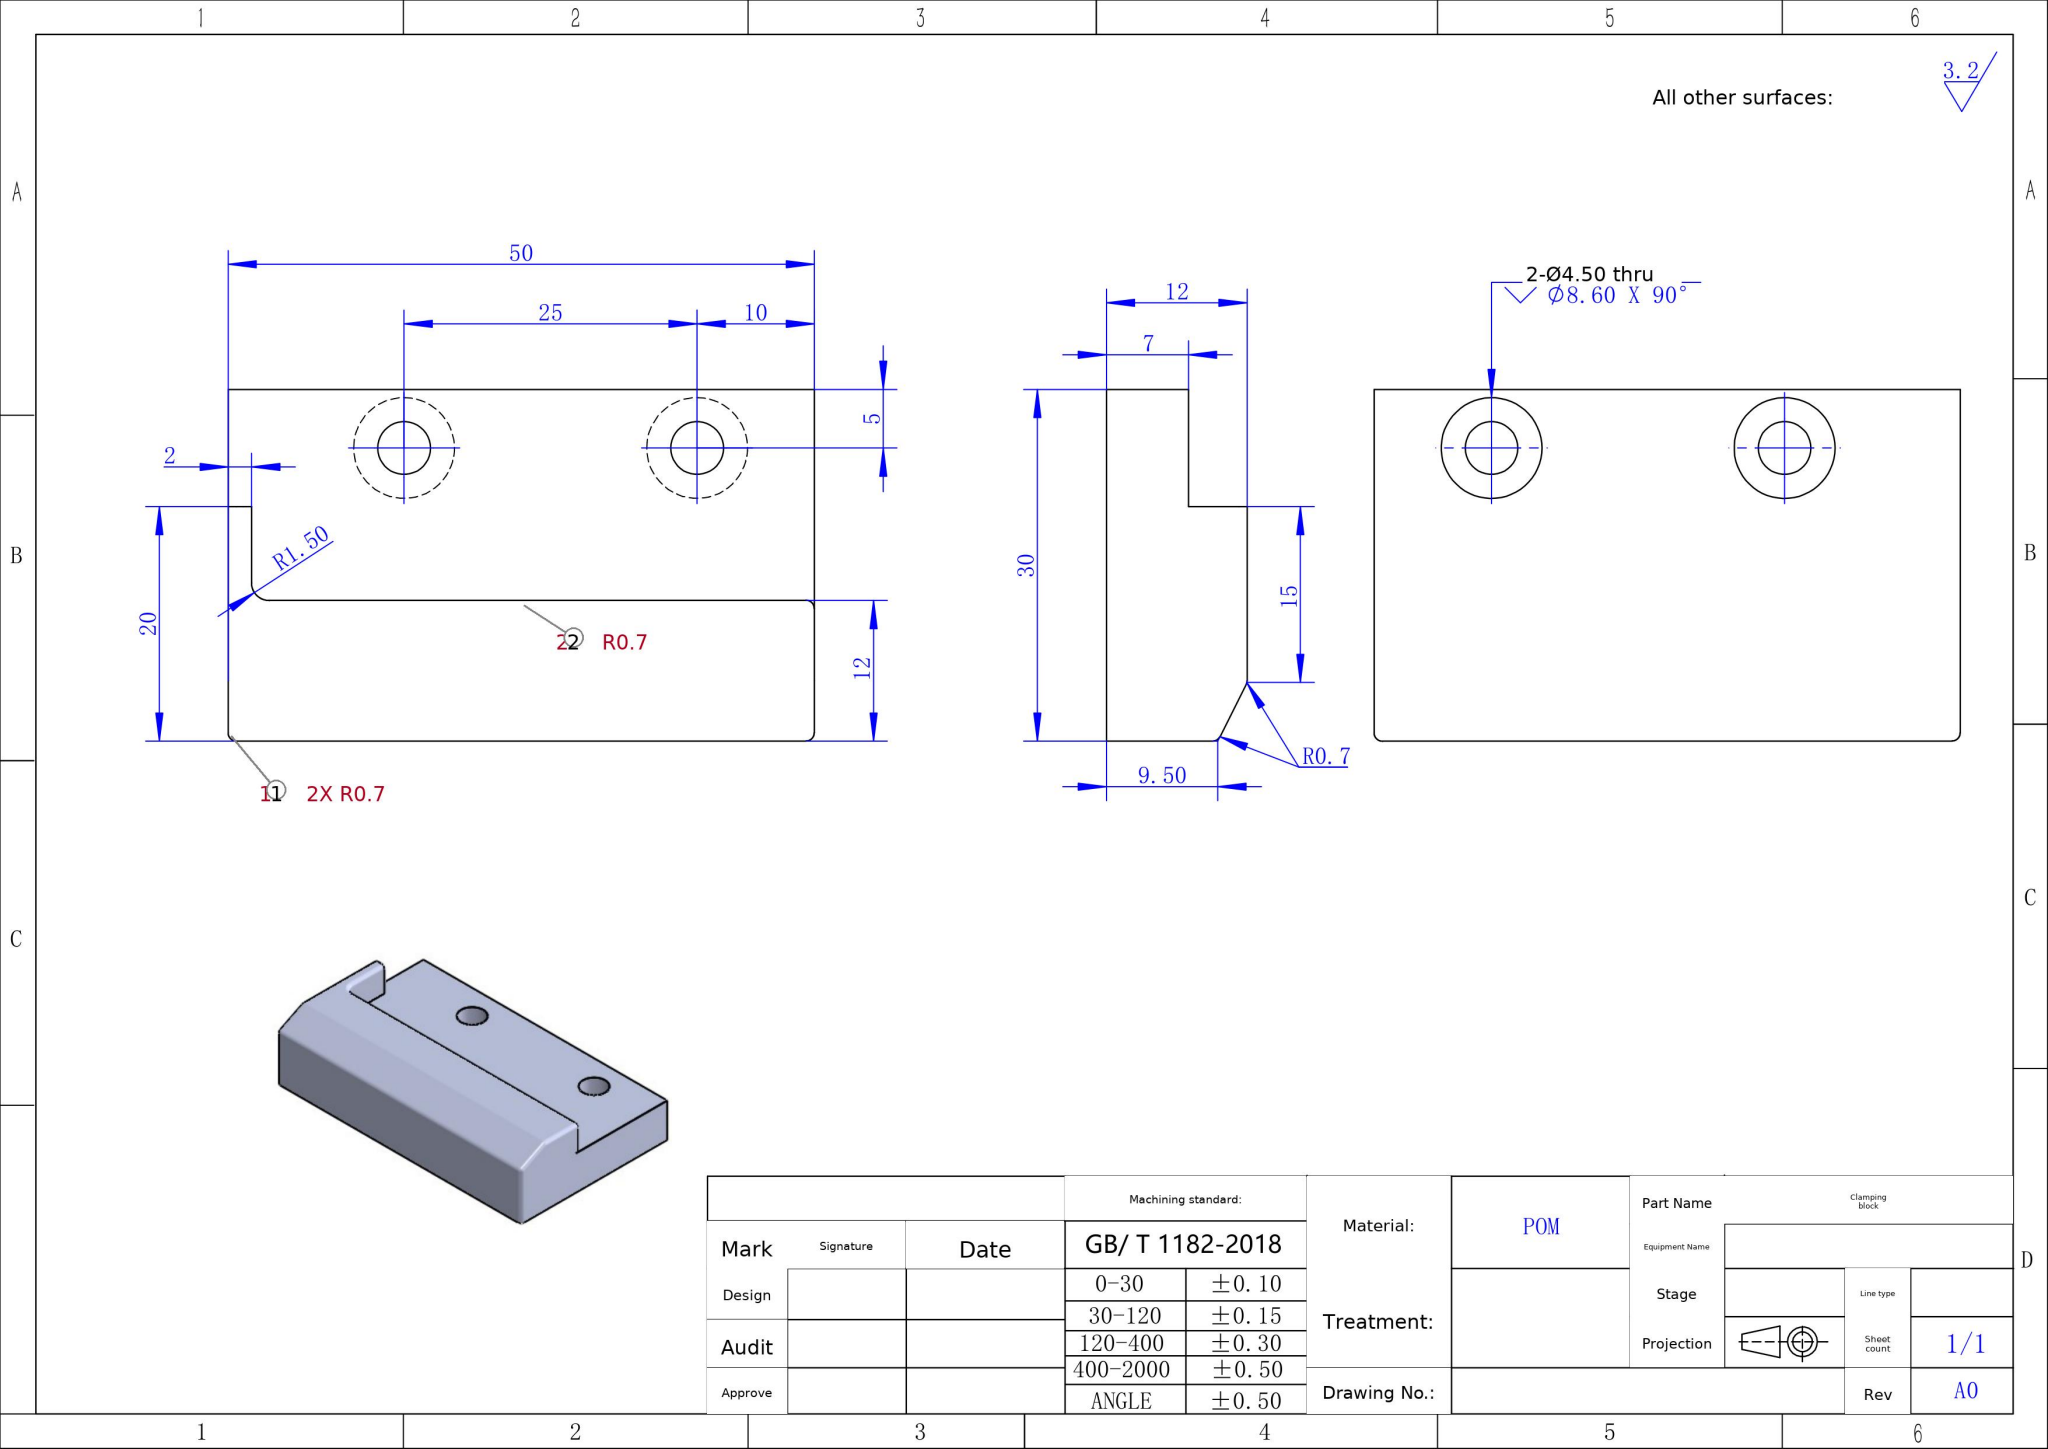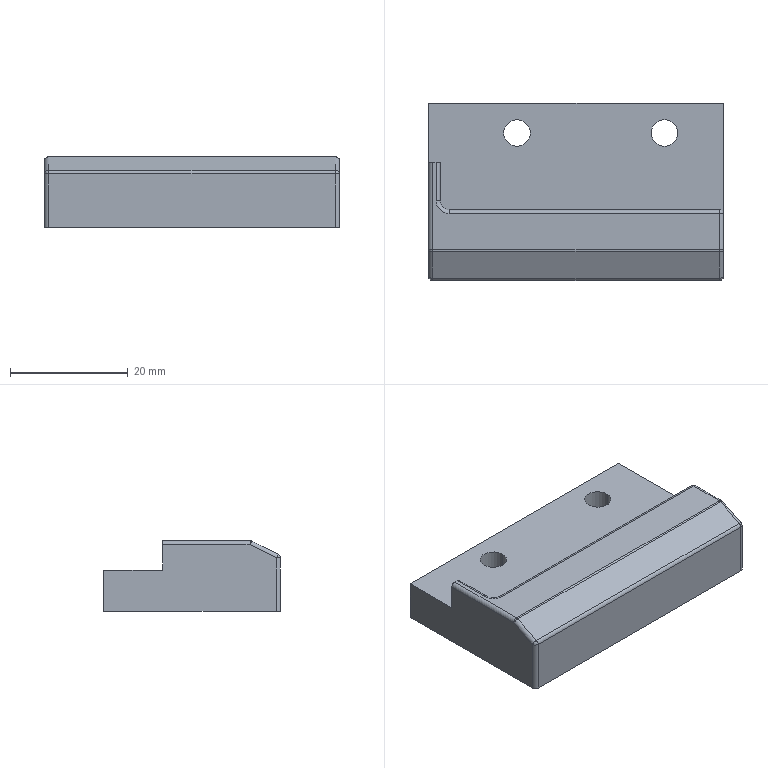Part | SolidWorks | mm | material POM | 1 solid | 37 faces | box 50 x 30 x 12 mm | volume 12956 mm3 | cylinder 16 | plane 11 | sphere 5 | cone 4 | torus 1 | commonest cylinder face diameters 1.4 x11 4.5 x4 3 x1
STEP:
#1=CARTESIAN_POINT('',(42.25,-5.,2.05));
#2=VERTEX_POINT('',#1);
#3=CARTESIAN_POINT('',(37.75,-5.,2.05));
#4=VERTEX_POINT('',#3);
#5=CARTESIAN_POINT('',(40.,-5.,2.05));
#6=DIRECTION('',(0.,0.,-1.));
#7=DIRECTION('',(-1.,0.,0.));
#8=AXIS2_PLACEMENT_3D('',#5,#6,#7);
#9=CIRCLE('',#8,2.25);
#10=EDGE_CURVE('',#2,#4,#9,.T.);
#11=ORIENTED_EDGE('',*,*,#10,.F.);
#12=CARTESIAN_POINT('',(44.3,-5.,0.));
#13=VERTEX_POINT('',#12);
#14=CARTESIAN_POINT('',(44.3,-5.,0.));
#15=DIRECTION('',(0.7071,0.,-0.7071));
#16=VECTOR('',#15,1000.);
#17=LINE('',#14,#16);
#18=EDGE_CURVE('',#2,#13,#17,.T.);
#19=ORIENTED_EDGE('',*,*,#18,.T.);
#20=CARTESIAN_POINT('',(35.7,-5.,0.));
#21=VERTEX_POINT('',#20);
#22=CARTESIAN_POINT('',(40.,-5.,0.));
#23=DIRECTION('',(0.,0.,-1.));
#24=DIRECTION('',(-1.,0.,0.));
#25=AXIS2_PLACEMENT_3D('',#22,#23,#24);
#26=CIRCLE('',#25,4.3);
#27=EDGE_CURVE('',#13,#21,#26,.T.);
#28=ORIENTED_EDGE('',*,*,#27,.T.);
#29=CARTESIAN_POINT('',(35.7,-5.,0.));
#30=DIRECTION('',(-0.7071,0.,-0.7071));
#31=VECTOR('',#30,1000.);
#32=LINE('',#29,#31);
#33=EDGE_CURVE('',#4,#21,#32,.T.);
#34=ORIENTED_EDGE('',*,*,#33,.F.);
#35=EDGE_LOOP('',(#11,#19,#28,#34));
#36=FACE_OUTER_BOUND('',#35,.T.);
#37=CARTESIAN_POINT('',(40.,-5.,0.));
#38=DIRECTION('',(0.,0.,-1.));
#39=DIRECTION('',(-1.,0.,0.));
#40=AXIS2_PLACEMENT_3D('',#37,#38,#39);
#41=CONICAL_SURFACE('',#40,4.3,0.7854);
#42=ADVANCED_FACE('',(#36),#41,.F.);
#43=CARTESIAN_POINT('',(42.25,-5.,7.));
#44=VERTEX_POINT('',#43);
#45=CARTESIAN_POINT('',(37.75,-5.,7.));
#46=VERTEX_POINT('',#45);
#47=CARTESIAN_POINT('',(40.,-5.,7.));
#48=DIRECTION('',(0.,0.,-1.));
#49=DIRECTION('',(-1.,0.,0.));
#50=AXIS2_PLACEMENT_3D('',#47,#48,#49);
#51=CIRCLE('',#50,2.25);
#52=EDGE_CURVE('',#44,#46,#51,.T.);
#53=ORIENTED_EDGE('',*,*,#52,.F.);
#54=CARTESIAN_POINT('',(42.25,-5.,0.));
#55=DIRECTION('',(0.,0.,-1.));
#56=VECTOR('',#55,1000.);
#57=LINE('',#54,#56);
#58=EDGE_CURVE('',#44,#2,#57,.T.);
#59=ORIENTED_EDGE('',*,*,#58,.T.);
#60=ORIENTED_EDGE('',*,*,#10,.T.);
#61=CARTESIAN_POINT('',(37.75,-5.,0.));
#62=DIRECTION('',(0.,0.,-1.));
#63=VECTOR('',#62,1000.);
#64=LINE('',#61,#63);
#65=EDGE_CURVE('',#46,#4,#64,.T.);
#66=ORIENTED_EDGE('',*,*,#65,.F.);
#67=EDGE_LOOP('',(#53,#59,#60,#66));
#68=FACE_OUTER_BOUND('',#67,.T.);
#69=CARTESIAN_POINT('',(40.,-5.,0.));
#70=DIRECTION('',(0.,0.,-1.));
#71=DIRECTION('',(-1.,0.,0.));
#72=AXIS2_PLACEMENT_3D('',#69,#70,#71);
#73=CYLINDRICAL_SURFACE('',#72,2.25);
#74=ADVANCED_FACE('',(#68),#73,.F.);
#75=CARTESIAN_POINT('',(17.25,-5.,2.05));
#76=VERTEX_POINT('',#75);
#77=CARTESIAN_POINT('',(12.75,-5.,2.05));
#78=VERTEX_POINT('',#77);
#79=CARTESIAN_POINT('',(15.,-5.,2.05));
#80=DIRECTION('',(0.,0.,-1.));
#81=DIRECTION('',(-1.,0.,0.));
#82=AXIS2_PLACEMENT_3D('',#79,#80,#81);
#83=CIRCLE('',#82,2.25);
#84=EDGE_CURVE('',#76,#78,#83,.T.);
#85=ORIENTED_EDGE('',*,*,#84,.F.);
#86=CARTESIAN_POINT('',(19.3,-5.,0.));
#87=VERTEX_POINT('',#86);
#88=CARTESIAN_POINT('',(19.3,-5.,0.));
#89=DIRECTION('',(0.7071,0.,-0.7071));
#90=VECTOR('',#89,1000.);
#91=LINE('',#88,#90);
#92=EDGE_CURVE('',#76,#87,#91,.T.);
#93=ORIENTED_EDGE('',*,*,#92,.T.);
#94=CARTESIAN_POINT('',(10.7,-5.,0.));
#95=VERTEX_POINT('',#94);
#96=CARTESIAN_POINT('',(15.,-5.,0.));
#97=DIRECTION('',(0.,0.,-1.));
#98=DIRECTION('',(-1.,0.,0.));
#99=AXIS2_PLACEMENT_3D('',#96,#97,#98);
#100=CIRCLE('',#99,4.3);
#101=EDGE_CURVE('',#87,#95,#100,.T.);
#102=ORIENTED_EDGE('',*,*,#101,.T.);
#103=CARTESIAN_POINT('',(10.7,-5.,0.));
#104=DIRECTION('',(-0.7071,0.,-0.7071));
#105=VECTOR('',#104,1000.);
#106=LINE('',#103,#105);
#107=EDGE_CURVE('',#78,#95,#106,.T.);
#108=ORIENTED_EDGE('',*,*,#107,.F.);
#109=EDGE_LOOP('',(#85,#93,#102,#108));
#110=FACE_OUTER_BOUND('',#109,.T.);
#111=CARTESIAN_POINT('',(15.,-5.,0.));
#112=DIRECTION('',(0.,0.,-1.));
#113=DIRECTION('',(-1.,0.,0.));
#114=AXIS2_PLACEMENT_3D('',#111,#112,#113);
#115=CONICAL_SURFACE('',#114,4.3,0.7854);
#116=ADVANCED_FACE('',(#110),#115,.F.);
#117=CARTESIAN_POINT('',(17.25,-5.,7.));
#118=VERTEX_POINT('',#117);
#119=CARTESIAN_POINT('',(12.75,-5.,7.));
#120=VERTEX_POINT('',#119);
#121=CARTESIAN_POINT('',(15.,-5.,7.));
#122=DIRECTION('',(0.,0.,-1.));
#123=DIRECTION('',(-1.,0.,0.));
#124=AXIS2_PLACEMENT_3D('',#121,#122,#123);
#125=CIRCLE('',#124,2.25);
#126=EDGE_CURVE('',#118,#120,#125,.T.);
#127=ORIENTED_EDGE('',*,*,#126,.F.);
#128=CARTESIAN_POINT('',(17.25,-5.,0.));
#129=DIRECTION('',(0.,0.,-1.));
#130=VECTOR('',#129,1000.);
#131=LINE('',#128,#130);
#132=EDGE_CURVE('',#118,#76,#131,.T.);
#133=ORIENTED_EDGE('',*,*,#132,.T.);
#134=ORIENTED_EDGE('',*,*,#84,.T.);
#135=CARTESIAN_POINT('',(12.75,-5.,0.));
#136=DIRECTION('',(0.,0.,-1.));
#137=VECTOR('',#136,1000.);
#138=LINE('',#135,#137);
#139=EDGE_CURVE('',#120,#78,#138,.T.);
#140=ORIENTED_EDGE('',*,*,#139,.F.);
#141=EDGE_LOOP('',(#127,#133,#134,#140));
#142=FACE_OUTER_BOUND('',#141,.T.);
#143=CARTESIAN_POINT('',(15.,-5.,0.));
#144=DIRECTION('',(0.,0.,-1.));
#145=DIRECTION('',(-1.,0.,0.));
#146=AXIS2_PLACEMENT_3D('',#143,#144,#145);
#147=CYLINDRICAL_SURFACE('',#146,2.25);
#148=ADVANCED_FACE('',(#142),#147,.F.);
#149=CARTESIAN_POINT('',(0.,0.,0.));
#150=VERTEX_POINT('',#149);
#151=CARTESIAN_POINT('',(0.,-29.3,0.));
#152=VERTEX_POINT('',#151);
#153=CARTESIAN_POINT('',(0.,0.,0.));
#154=DIRECTION('',(0.,-1.,0.));
#155=VECTOR('',#154,1000.);
#156=LINE('',#153,#155);
#157=EDGE_CURVE('',#150,#152,#156,.T.);
#158=ORIENTED_EDGE('',*,*,#157,.T.);
#159=CARTESIAN_POINT('',(0.,-29.3,9.067));
#160=VERTEX_POINT('',#159);
#161=CARTESIAN_POINT('',(0.,-29.3,12.));
#162=DIRECTION('',(0.,0.,1.));
#163=VECTOR('',#162,1000.);
#164=LINE('',#161,#163);
#165=EDGE_CURVE('',#152,#160,#164,.T.);
#166=ORIENTED_EDGE('',*,*,#165,.T.);
#167=CARTESIAN_POINT('',(0.,-24.835,11.3));
#168=VERTEX_POINT('',#167);
#169=CARTESIAN_POINT('',(0.,-4.687,21.374));
#170=DIRECTION('',(-0.,0.8944,0.4472));
#171=VECTOR('',#170,1000.);
#172=LINE('',#169,#171);
#173=EDGE_CURVE('',#160,#168,#172,.T.);
#174=ORIENTED_EDGE('',*,*,#173,.T.);
#175=CARTESIAN_POINT('',(0.,-10.,11.3));
#176=VERTEX_POINT('',#175);
#177=CARTESIAN_POINT('',(0.,-10.,11.3));
#178=DIRECTION('',(-0.,1.,0.));
#179=VECTOR('',#178,1000.);
#180=LINE('',#177,#179);
#181=EDGE_CURVE('',#168,#176,#180,.T.);
#182=ORIENTED_EDGE('',*,*,#181,.T.);
#183=CARTESIAN_POINT('',(0.,-10.,7.));
#184=VERTEX_POINT('',#183);
#185=CARTESIAN_POINT('',(0.,-10.,12.));
#186=DIRECTION('',(0.,0.,-1.));
#187=VECTOR('',#186,1000.);
#188=LINE('',#185,#187);
#189=EDGE_CURVE('',#176,#184,#188,.T.);
#190=ORIENTED_EDGE('',*,*,#189,.T.);
#191=CARTESIAN_POINT('',(0.,0.,7.));
#192=VERTEX_POINT('',#191);
#193=CARTESIAN_POINT('',(0.,0.,7.));
#194=DIRECTION('',(-0.,1.,0.));
#195=VECTOR('',#194,1000.);
#196=LINE('',#193,#195);
#197=EDGE_CURVE('',#184,#192,#196,.T.);
#198=ORIENTED_EDGE('',*,*,#197,.T.);
#199=CARTESIAN_POINT('',(0.,0.,12.));
#200=DIRECTION('',(0.,0.,-1.));
#201=VECTOR('',#200,1000.);
#202=LINE('',#199,#201);
#203=EDGE_CURVE('',#192,#150,#202,.T.);
#204=ORIENTED_EDGE('',*,*,#203,.T.);
#205=EDGE_LOOP('',(#158,#166,#174,#182,#190,#198,#204));
#206=FACE_OUTER_BOUND('',#205,.T.);
#207=CARTESIAN_POINT('',(0.,0.,12.));
#208=DIRECTION('',(1.,0.,0.));
#209=DIRECTION('',(-0.,1.,0.));
#210=AXIS2_PLACEMENT_3D('',#207,#208,#209);
#211=PLANE('',#210);
#212=ADVANCED_FACE('',(#206),#211,.F.);
#213=CARTESIAN_POINT('',(0.7,-30.,0.));
#214=VERTEX_POINT('',#213);
#215=CARTESIAN_POINT('',(49.3,-30.,0.));
#216=VERTEX_POINT('',#215);
#217=CARTESIAN_POINT('',(0.,-30.,0.));
#218=DIRECTION('',(1.,0.,0.));
#219=VECTOR('',#218,1000.);
#220=LINE('',#217,#219);
#221=EDGE_CURVE('',#214,#216,#220,.T.);
#222=ORIENTED_EDGE('',*,*,#221,.T.);
#223=CARTESIAN_POINT('',(49.3,-30.,9.067));
#224=VERTEX_POINT('',#223);
#225=CARTESIAN_POINT('',(49.3,-30.,12.));
#226=DIRECTION('',(0.,0.,1.));
#227=VECTOR('',#226,1000.);
#228=LINE('',#225,#227);
#229=EDGE_CURVE('',#216,#224,#228,.T.);
#230=ORIENTED_EDGE('',*,*,#229,.T.);
#231=CARTESIAN_POINT('',(0.7,-30.,9.067));
#232=VERTEX_POINT('',#231);
#233=CARTESIAN_POINT('',(0.,-30.,9.067));
#234=DIRECTION('',(-1.,0.,0.));
#235=VECTOR('',#234,1000.);
#236=LINE('',#233,#235);
#237=EDGE_CURVE('',#224,#232,#236,.T.);
#238=ORIENTED_EDGE('',*,*,#237,.T.);
#239=CARTESIAN_POINT('',(0.7,-30.,12.));
#240=DIRECTION('',(0.,0.,-1.));
#241=VECTOR('',#240,1000.);
#242=LINE('',#239,#241);
#243=EDGE_CURVE('',#232,#214,#242,.T.);
#244=ORIENTED_EDGE('',*,*,#243,.T.);
#245=EDGE_LOOP('',(#222,#230,#238,#244));
#246=FACE_OUTER_BOUND('',#245,.T.);
#247=CARTESIAN_POINT('',(0.,-30.,12.));
#248=DIRECTION('',(0.,1.,0.));
#249=DIRECTION('',(0.,0.,1.));
#250=AXIS2_PLACEMENT_3D('',#247,#248,#249);
#251=PLANE('',#250);
#252=ADVANCED_FACE('',(#246),#251,.F.);
#253=CARTESIAN_POINT('',(50.,0.,7.));
#254=VERTEX_POINT('',#253);
#255=CARTESIAN_POINT('',(50.,-18.7,7.));
#256=VERTEX_POINT('',#255);
#257=CARTESIAN_POINT('',(50.,0.,7.));
#258=DIRECTION('',(0.,-1.,0.));
#259=VECTOR('',#258,1000.);
#260=LINE('',#257,#259);
#261=EDGE_CURVE('',#254,#256,#260,.T.);
#262=ORIENTED_EDGE('',*,*,#261,.T.);
#263=CARTESIAN_POINT('',(50.,-18.7,11.3));
#264=VERTEX_POINT('',#263);
#265=CARTESIAN_POINT('',(50.,-18.7,12.));
#266=DIRECTION('',(0.,0.,1.));
#267=VECTOR('',#266,1000.);
#268=LINE('',#265,#267);
#269=EDGE_CURVE('',#256,#264,#268,.T.);
#270=ORIENTED_EDGE('',*,*,#269,.T.);
#271=CARTESIAN_POINT('',(50.,-24.835,11.3));
#272=VERTEX_POINT('',#271);
#273=CARTESIAN_POINT('',(50.,-25.,11.3));
#274=DIRECTION('',(0.,-1.,0.));
#275=VECTOR('',#274,1000.);
#276=LINE('',#273,#275);
#277=EDGE_CURVE('',#264,#272,#276,.T.);
#278=ORIENTED_EDGE('',*,*,#277,.T.);
#279=CARTESIAN_POINT('',(50.,-29.3,9.067));
#280=VERTEX_POINT('',#279);
#281=CARTESIAN_POINT('',(50.,-4.687,21.374));
#282=DIRECTION('',(0.,-0.8944,-0.4472));
#283=VECTOR('',#282,1000.);
#284=LINE('',#281,#283);
#285=EDGE_CURVE('',#272,#280,#284,.T.);
#286=ORIENTED_EDGE('',*,*,#285,.T.);
#287=CARTESIAN_POINT('',(50.,-29.3,0.));
#288=VERTEX_POINT('',#287);
#289=CARTESIAN_POINT('',(50.,-29.3,12.));
#290=DIRECTION('',(0.,0.,-1.));
#291=VECTOR('',#290,1000.);
#292=LINE('',#289,#291);
#293=EDGE_CURVE('',#280,#288,#292,.T.);
#294=ORIENTED_EDGE('',*,*,#293,.T.);
#295=CARTESIAN_POINT('',(50.,0.,0.));
#296=VERTEX_POINT('',#295);
#297=CARTESIAN_POINT('',(50.,0.,0.));
#298=DIRECTION('',(-0.,1.,0.));
#299=VECTOR('',#298,1000.);
#300=LINE('',#297,#299);
#301=EDGE_CURVE('',#288,#296,#300,.T.);
#302=ORIENTED_EDGE('',*,*,#301,.T.);
#303=CARTESIAN_POINT('',(50.,0.,12.));
#304=DIRECTION('',(0.,0.,-1.));
#305=VECTOR('',#304,1000.);
#306=LINE('',#303,#305);
#307=EDGE_CURVE('',#254,#296,#306,.T.);
#308=ORIENTED_EDGE('',*,*,#307,.F.);
#309=EDGE_LOOP('',(#262,#270,#278,#286,#294,#302,#308));
#310=FACE_OUTER_BOUND('',#309,.T.);
#311=CARTESIAN_POINT('',(50.,0.,12.));
#312=DIRECTION('',(-1.,-0.,0.));
#313=DIRECTION('',(0.,-1.,0.));
#314=AXIS2_PLACEMENT_3D('',#311,#312,#313);
#315=PLANE('',#314);
#316=ADVANCED_FACE('',(#310),#315,.F.);
#317=ORIENTED_EDGE('',*,*,#203,.F.);
#318=CARTESIAN_POINT('',(0.,0.,7.));
#319=DIRECTION('',(1.,0.,0.));
#320=VECTOR('',#319,1000.);
#321=LINE('',#318,#320);
#322=EDGE_CURVE('',#192,#254,#321,.T.);
#323=ORIENTED_EDGE('',*,*,#322,.T.);
#324=ORIENTED_EDGE('',*,*,#307,.T.);
#325=CARTESIAN_POINT('',(0.,0.,0.));
#326=DIRECTION('',(-1.,0.,0.));
#327=VECTOR('',#326,1000.);
#328=LINE('',#325,#327);
#329=EDGE_CURVE('',#296,#150,#328,.T.);
#330=ORIENTED_EDGE('',*,*,#329,.T.);
#331=EDGE_LOOP('',(#317,#323,#324,#330));
#332=FACE_OUTER_BOUND('',#331,.T.);
#333=CARTESIAN_POINT('',(0.,0.,12.));
#334=DIRECTION('',(0.,-1.,0.));
#335=DIRECTION('',(0.,0.,-1.));
#336=AXIS2_PLACEMENT_3D('',#333,#334,#335);
#337=PLANE('',#336);
#338=ADVANCED_FACE('',(#332),#337,.F.);
#339=CARTESIAN_POINT('',(0.7,-10.,12.));
#340=VERTEX_POINT('',#339);
#341=CARTESIAN_POINT('',(1.3,-10.,12.));
#342=VERTEX_POINT('',#341);
#343=CARTESIAN_POINT('',(0.,-10.,12.));
#344=DIRECTION('',(1.,0.,0.));
#345=VECTOR('',#344,1000.);
#346=LINE('',#343,#345);
#347=EDGE_CURVE('',#340,#342,#346,.T.);
#348=ORIENTED_EDGE('',*,*,#347,.F.);
#349=CARTESIAN_POINT('',(0.7,-24.835,12.));
#350=VERTEX_POINT('',#349);
#351=CARTESIAN_POINT('',(0.7,-25.,12.));
#352=DIRECTION('',(0.,-1.,0.));
#353=VECTOR('',#352,1000.);
#354=LINE('',#351,#353);
#355=EDGE_CURVE('',#340,#350,#354,.T.);
#356=ORIENTED_EDGE('',*,*,#355,.T.);
#357=CARTESIAN_POINT('',(49.3,-24.835,12.));
#358=VERTEX_POINT('',#357);
#359=CARTESIAN_POINT('',(50.,-24.835,12.));
#360=DIRECTION('',(1.,0.,0.));
#361=VECTOR('',#360,1000.);
#362=LINE('',#359,#361);
#363=EDGE_CURVE('',#350,#358,#362,.T.);
#364=ORIENTED_EDGE('',*,*,#363,.T.);
#365=CARTESIAN_POINT('',(49.3,-18.7,12.));
#366=VERTEX_POINT('',#365);
#367=CARTESIAN_POINT('',(49.3,-18.,12.));
#368=DIRECTION('',(-0.,1.,0.));
#369=VECTOR('',#368,1000.);
#370=LINE('',#367,#369);
#371=EDGE_CURVE('',#358,#366,#370,.T.);
#372=ORIENTED_EDGE('',*,*,#371,.T.);
#373=CARTESIAN_POINT('',(3.5,-18.7,12.));
#374=VERTEX_POINT('',#373);
#375=CARTESIAN_POINT('',(3.5,-18.7,12.));
#376=DIRECTION('',(-1.,0.,0.));
#377=VECTOR('',#376,1000.);
#378=LINE('',#375,#377);
#379=EDGE_CURVE('',#366,#374,#378,.T.);
#380=ORIENTED_EDGE('',*,*,#379,.T.);
#381=CARTESIAN_POINT('',(1.3,-16.5,12.));
#382=VERTEX_POINT('',#381);
#383=CARTESIAN_POINT('',(3.5,-16.5,12.));
#384=DIRECTION('',(0.,0.,-1.));
#385=DIRECTION('',(1.,0.,0.));
#386=AXIS2_PLACEMENT_3D('',#383,#384,#385);
#387=CIRCLE('',#386,2.2);
#388=EDGE_CURVE('',#374,#382,#387,.T.);
#389=ORIENTED_EDGE('',*,*,#388,.T.);
#390=CARTESIAN_POINT('',(1.3,-10.,12.));
#391=DIRECTION('',(-0.,1.,0.));
#392=VECTOR('',#391,1000.);
#393=LINE('',#390,#392);
#394=EDGE_CURVE('',#382,#342,#393,.T.);
#395=ORIENTED_EDGE('',*,*,#394,.T.);
#396=EDGE_LOOP('',(#348,#356,#364,#372,#380,#389,#395));
#397=FACE_OUTER_BOUND('',#396,.T.);
#398=CARTESIAN_POINT('',(0.,0.,12.));
#399=DIRECTION('',(0.,0.,1.));
#400=DIRECTION('',(1.,0.,0.));
#401=AXIS2_PLACEMENT_3D('',#398,#399,#400);
#402=PLANE('',#401);
#403=ADVANCED_FACE('',(#397),#402,.T.);
#404=CARTESIAN_POINT('',(40.,-5.,0.));
#405=DIRECTION('',(0.,0.,-1.));
#406=DIRECTION('',(-1.,0.,0.));
#407=AXIS2_PLACEMENT_3D('',#404,#405,#406);
#408=CIRCLE('',#407,4.3);
#409=EDGE_CURVE('',#21,#13,#408,.T.);
#410=ORIENTED_EDGE('',*,*,#409,.F.);
#411=ORIENTED_EDGE('',*,*,#27,.F.);
#412=EDGE_LOOP('',(#410,#411));
#413=FACE_BOUND('',#412,.T.);
#414=CARTESIAN_POINT('',(15.,-5.,0.));
#415=DIRECTION('',(0.,0.,-1.));
#416=DIRECTION('',(-1.,0.,0.));
#417=AXIS2_PLACEMENT_3D('',#414,#415,#416);
#418=CIRCLE('',#417,4.3);
#419=EDGE_CURVE('',#95,#87,#418,.T.);
#420=ORIENTED_EDGE('',*,*,#419,.F.);
#421=ORIENTED_EDGE('',*,*,#101,.F.);
#422=EDGE_LOOP('',(#420,#421));
#423=FACE_BOUND('',#422,.T.);
#424=ORIENTED_EDGE('',*,*,#301,.F.);
#425=CARTESIAN_POINT('',(49.3,-29.3,0.));
#426=DIRECTION('',(0.,0.,-1.));
#427=DIRECTION('',(1.,0.,0.));
#428=AXIS2_PLACEMENT_3D('',#425,#426,#427);
#429=CIRCLE('',#428,0.7);
#430=EDGE_CURVE('',#288,#216,#429,.T.);
#431=ORIENTED_EDGE('',*,*,#430,.T.);
#432=ORIENTED_EDGE('',*,*,#221,.F.);
#433=CARTESIAN_POINT('',(0.7,-29.3,0.));
#434=DIRECTION('',(0.,0.,-1.));
#435=DIRECTION('',(1.,0.,0.));
#436=AXIS2_PLACEMENT_3D('',#433,#434,#435);
#437=CIRCLE('',#436,0.7);
#438=EDGE_CURVE('',#214,#152,#437,.T.);
#439=ORIENTED_EDGE('',*,*,#438,.T.);
#440=ORIENTED_EDGE('',*,*,#157,.F.);
#441=ORIENTED_EDGE('',*,*,#329,.F.);
#442=EDGE_LOOP('',(#424,#431,#432,#439,#440,#441));
#443=FACE_OUTER_BOUND('',#442,.T.);
#444=CARTESIAN_POINT('',(0.,0.,0.));
#445=DIRECTION('',(0.,0.,1.));
#446=DIRECTION('',(1.,0.,0.));
#447=AXIS2_PLACEMENT_3D('',#444,#445,#446);
#448=PLANE('',#447);
#449=ADVANCED_FACE('',(#413,#423,#443),#448,.F.);
#450=CARTESIAN_POINT('',(40.,-5.,7.));
#451=DIRECTION('',(0.,0.,-1.));
#452=DIRECTION('',(-1.,0.,0.));
#453=AXIS2_PLACEMENT_3D('',#450,#451,#452);
#454=CIRCLE('',#453,2.25);
#455=EDGE_CURVE('',#46,#44,#454,.T.);
#456=ORIENTED_EDGE('',*,*,#455,.T.);
#457=ORIENTED_EDGE('',*,*,#52,.T.);
#458=EDGE_LOOP('',(#456,#457));
#459=FACE_BOUND('',#458,.T.);
#460=CARTESIAN_POINT('',(15.,-5.,7.));
#461=DIRECTION('',(0.,0.,-1.));
#462=DIRECTION('',(-1.,0.,0.));
#463=AXIS2_PLACEMENT_3D('',#460,#461,#462);
#464=CIRCLE('',#463,2.25);
#465=EDGE_CURVE('',#120,#118,#464,.T.);
#466=ORIENTED_EDGE('',*,*,#465,.T.);
#467=ORIENTED_EDGE('',*,*,#126,.T.);
#468=EDGE_LOOP('',(#466,#467));
#469=FACE_BOUND('',#468,.T.);
#470=CARTESIAN_POINT('',(2.,-10.,7.));
#471=VERTEX_POINT('',#470);
#472=CARTESIAN_POINT('',(2.,-16.5,7.));
#473=VERTEX_POINT('',#472);
#474=CARTESIAN_POINT('',(2.,-10.,7.));
#475=DIRECTION('',(0.,-1.,0.));
#476=VECTOR('',#475,1000.);
#477=LINE('',#474,#476);
#478=EDGE_CURVE('',#471,#473,#477,.T.);
#479=ORIENTED_EDGE('',*,*,#478,.T.);
#480=CARTESIAN_POINT('',(3.5,-18.,7.));
#481=VERTEX_POINT('',#480);
#482=CARTESIAN_POINT('',(3.5,-16.5,7.));
#483=DIRECTION('',(0.,0.,1.));
#484=DIRECTION('',(-1.,0.,0.));
#485=AXIS2_PLACEMENT_3D('',#482,#483,#484);
#486=CIRCLE('',#485,1.5);
#487=EDGE_CURVE('',#473,#481,#486,.T.);
#488=ORIENTED_EDGE('',*,*,#487,.T.);
#489=CARTESIAN_POINT('',(49.3,-18.,7.));
#490=VERTEX_POINT('',#489);
#491=CARTESIAN_POINT('',(2.,-18.,7.));
#492=DIRECTION('',(1.,0.,0.));
#493=VECTOR('',#492,1000.);
#494=LINE('',#491,#493);
#495=EDGE_CURVE('',#481,#490,#494,.T.);
#496=ORIENTED_EDGE('',*,*,#495,.T.);
#497=CARTESIAN_POINT('',(49.3,-18.7,7.));
#498=DIRECTION('',(0.,0.,-1.));
#499=DIRECTION('',(-1.,0.,0.));
#500=AXIS2_PLACEMENT_3D('',#497,#498,#499);
#501=CIRCLE('',#500,0.7);
#502=EDGE_CURVE('',#490,#256,#501,.T.);
#503=ORIENTED_EDGE('',*,*,#502,.T.);
#504=ORIENTED_EDGE('',*,*,#261,.F.);
#505=ORIENTED_EDGE('',*,*,#322,.F.);
#506=ORIENTED_EDGE('',*,*,#197,.F.);
#507=CARTESIAN_POINT('',(-4.226,-10.,7.));
#508=DIRECTION('',(1.,0.,0.));
#509=VECTOR('',#508,1000.);
#510=LINE('',#507,#509);
#511=EDGE_CURVE('',#184,#471,#510,.T.);
#512=ORIENTED_EDGE('',*,*,#511,.T.);
#513=EDGE_LOOP('',(#479,#488,#496,#503,#504,#505,#506,#512));
#514=FACE_OUTER_BOUND('',#513,.T.);
#515=CARTESIAN_POINT('',(0.,0.,7.));
#516=DIRECTION('',(0.,0.,-1.));
#517=DIRECTION('',(-1.,0.,0.));
#518=AXIS2_PLACEMENT_3D('',#515,#516,#517);
#519=PLANE('',#518);
#520=ADVANCED_FACE('',(#459,#469,#514),#519,.F.);
#521=CARTESIAN_POINT('',(3.5,-18.,11.3));
#522=VERTEX_POINT('',#521);
#523=CARTESIAN_POINT('',(3.5,-18.,12.));
#524=DIRECTION('',(0.,0.,1.));
#525=VECTOR('',#524,1000.);
#526=LINE('',#523,#525);
#527=EDGE_CURVE('',#481,#522,#526,.T.);
#528=ORIENTED_EDGE('',*,*,#527,.T.);
#529=CARTESIAN_POINT('',(49.3,-18.,11.3));
#530=VERTEX_POINT('',#529);
#531=CARTESIAN_POINT('',(50.,-18.,11.3));
#532=DIRECTION('',(1.,0.,0.));
#533=VECTOR('',#532,1000.);
#534=LINE('',#531,#533);
#535=EDGE_CURVE('',#522,#530,#534,.T.);
#536=ORIENTED_EDGE('',*,*,#535,.T.);
#537=CARTESIAN_POINT('',(49.3,-18.,7.));
#538=DIRECTION('',(0.,0.,-1.));
#539=VECTOR('',#538,1000.);
#540=LINE('',#537,#539);
#541=EDGE_CURVE('',#530,#490,#540,.T.);
#542=ORIENTED_EDGE('',*,*,#541,.T.);
#543=ORIENTED_EDGE('',*,*,#495,.F.);
#544=EDGE_LOOP('',(#528,#536,#542,#543));
#545=FACE_OUTER_BOUND('',#544,.T.);
#546=CARTESIAN_POINT('',(2.,-18.,7.));
#547=DIRECTION('',(0.,-1.,0.));
#548=DIRECTION('',(0.,0.,-1.));
#549=AXIS2_PLACEMENT_3D('',#546,#547,#548);
#550=PLANE('',#549);
#551=ADVANCED_FACE('',(#545),#550,.F.);
#552=ORIENTED_EDGE('',*,*,#189,.F.);
#553=CARTESIAN_POINT('',(0.7,-10.,11.3));
#554=DIRECTION('',(0.,1.,0.));
#555=DIRECTION('',(0.,0.,-1.));
#556=AXIS2_PLACEMENT_3D('',#553,#554,#555);
#557=CIRCLE('',#556,0.7);
#558=EDGE_CURVE('',#176,#340,#557,.T.);
#559=ORIENTED_EDGE('',*,*,#558,.T.);
#560=ORIENTED_EDGE('',*,*,#347,.T.);
#561=CARTESIAN_POINT('',(2.,-10.,11.3));
#562=VERTEX_POINT('',#561);
#563=CARTESIAN_POINT('',(1.3,-10.,11.3));
#564=DIRECTION('',(0.,1.,0.));
#565=DIRECTION('',(0.,0.,-1.));
#566=AXIS2_PLACEMENT_3D('',#563,#564,#565);
#567=CIRCLE('',#566,0.7);
#568=EDGE_CURVE('',#342,#562,#567,.T.);
#569=ORIENTED_EDGE('',*,*,#568,.T.);
#570=CARTESIAN_POINT('',(2.,-10.,7.));
#571=DIRECTION('',(0.,0.,1.));
#572=VECTOR('',#571,1000.);
#573=LINE('',#570,#572);
#574=EDGE_CURVE('',#471,#562,#573,.T.);
#575=ORIENTED_EDGE('',*,*,#574,.F.);
#576=ORIENTED_EDGE('',*,*,#511,.F.);
#577=EDGE_LOOP('',(#552,#559,#560,#569,#575,#576));
#578=FACE_OUTER_BOUND('',#577,.T.);
#579=CARTESIAN_POINT('',(-4.226,-10.,7.));
#580=DIRECTION('',(0.,-1.,0.));
#581=DIRECTION('',(0.,0.,-1.));
#582=AXIS2_PLACEMENT_3D('',#579,#580,#581);
#583=PLANE('',#582);
#584=ADVANCED_FACE('',(#578),#583,.F.);
#585=ORIENTED_EDGE('',*,*,#574,.T.);
#586=CARTESIAN_POINT('',(2.,-16.5,11.3));
#587=VERTEX_POINT('',#586);
#588=CARTESIAN_POINT('',(2.,-16.5,11.3));
#589=DIRECTION('',(0.,-1.,0.));
#590=VECTOR('',#589,1000.);
#591=LINE('',#588,#590);
#592=EDGE_CURVE('',#562,#587,#591,.T.);
#593=ORIENTED_EDGE('',*,*,#592,.T.);
#594=CARTESIAN_POINT('',(2.,-16.5,7.));
#595=DIRECTION('',(0.,0.,-1.));
#596=VECTOR('',#595,1000.);
#597=LINE('',#594,#596);
#598=EDGE_CURVE('',#587,#473,#597,.T.);
#599=ORIENTED_EDGE('',*,*,#598,.T.);
#600=ORIENTED_EDGE('',*,*,#478,.F.);
#601=EDGE_LOOP('',(#585,#593,#599,#600));
#602=FACE_OUTER_BOUND('',#601,.T.);
#603=CARTESIAN_POINT('',(2.,-10.,7.));
#604=DIRECTION('',(-1.,-0.,0.));
#605=DIRECTION('',(0.,-1.,0.));
#606=AXIS2_PLACEMENT_3D('',#603,#604,#605);
#607=PLANE('',#606);
#608=ADVANCED_FACE('',(#602),#607,.F.);
#609=ORIENTED_EDGE('',*,*,#598,.F.);
#610=CARTESIAN_POINT('',(3.5,-16.5,11.3));
#611=DIRECTION('',(0.,0.,1.));
#612=DIRECTION('',(1.,0.,0.));
#613=AXIS2_PLACEMENT_3D('',#610,#611,#612);
#614=CIRCLE('',#613,1.5);
#615=EDGE_CURVE('',#587,#522,#614,.T.);
#616=ORIENTED_EDGE('',*,*,#615,.T.);
#617=ORIENTED_EDGE('',*,*,#527,.F.);
#618=ORIENTED_EDGE('',*,*,#487,.F.);
#619=EDGE_LOOP('',(#609,#616,#617,#618));
#620=FACE_OUTER_BOUND('',#619,.T.);
#621=CARTESIAN_POINT('',(3.5,-16.5,7.));
#622=DIRECTION('',(0.,0.,-1.));
#623=DIRECTION('',(-1.,0.,0.));
#624=AXIS2_PLACEMENT_3D('',#621,#622,#623);
#625=CYLINDRICAL_SURFACE('',#624,1.5);
#626=ADVANCED_FACE('',(#620),#625,.F.);
#627=CARTESIAN_POINT('',(0.7,-29.613,9.693));
#628=VERTEX_POINT('',#627);
#629=CARTESIAN_POINT('',(49.3,-29.613,9.693));
#630=VERTEX_POINT('',#629);
#631=CARTESIAN_POINT('',(50.,-29.613,9.693));
#632=DIRECTION('',(1.,0.,-0.));
#633=VECTOR('',#632,1000.);
#634=LINE('',#631,#633);
#635=EDGE_CURVE('',#628,#630,#634,.T.);
#636=ORIENTED_EDGE('',*,*,#635,.T.);
#637=CARTESIAN_POINT('',(49.3,-25.148,11.926));
#638=VERTEX_POINT('',#637);
#639=CARTESIAN_POINT('',(49.3,-30.,9.5));
#640=DIRECTION('',(-0.,0.8944,0.4472));
#641=VECTOR('',#640,1000.);
#642=LINE('',#639,#641);
#643=EDGE_CURVE('',#630,#638,#642,.T.);
#644=ORIENTED_EDGE('',*,*,#643,.T.);
#645=CARTESIAN_POINT('',(0.7,-25.148,11.926));
#646=VERTEX_POINT('',#645);
#647=CARTESIAN_POINT('',(0.,-25.148,11.926));
#648=DIRECTION('',(-1.,-0.,0.));
#649=VECTOR('',#648,1000.);
#650=LINE('',#647,#649);
#651=EDGE_CURVE('',#638,#646,#650,.T.);
#652=ORIENTED_EDGE('',*,*,#651,.T.);
#653=CARTESIAN_POINT('',(0.7,-30.,9.5));
#654=DIRECTION('',(0.,-0.8944,-0.4472));
#655=VECTOR('',#654,1000.);
#656=LINE('',#653,#655);
#657=EDGE_CURVE('',#646,#628,#656,.T.);
#658=ORIENTED_EDGE('',*,*,#657,.T.);
#659=EDGE_LOOP('',(#636,#644,#652,#658));
#660=FACE_OUTER_BOUND('',#659,.T.);
#661=CARTESIAN_POINT('',(50.,-30.,9.5));
#662=DIRECTION('',(-0.,0.4472,-0.8944));
#663=DIRECTION('',(0.,0.8944,0.4472));
#664=AXIS2_PLACEMENT_3D('',#661,#662,#663);
#665=PLANE('',#664);
#666=ADVANCED_FACE('',(#660),#665,.F.);
#667=CARTESIAN_POINT('',(0.7,-29.3,9.067));
#668=DIRECTION('',(0.,0.,1.));
#669=DIRECTION('',(1.,0.,0.));
#670=AXIS2_PLACEMENT_3D('',#667,#668,#669);
#671=CIRCLE('',#670,0.7);
#672=EDGE_CURVE('',#160,#232,#671,.T.);
#673=ORIENTED_EDGE('',*,*,#672,.F.);
#674=ORIENTED_EDGE('',*,*,#165,.F.);
#675=ORIENTED_EDGE('',*,*,#438,.F.);
#676=ORIENTED_EDGE('',*,*,#243,.F.);
#677=EDGE_LOOP('',(#673,#674,#675,#676));
#678=FACE_OUTER_BOUND('',#677,.T.);
#679=CARTESIAN_POINT('',(0.7,-29.3,12.));
#680=DIRECTION('',(0.,0.,-1.));
#681=DIRECTION('',(-1.,0.,0.));
#682=AXIS2_PLACEMENT_3D('',#679,#680,#681);
#683=CYLINDRICAL_SURFACE('',#682,0.7);
#684=ADVANCED_FACE('',(#678),#683,.T.);
#685=CARTESIAN_POINT('',(0.7,-29.3,9.067));
#686=DIRECTION('',(0.,0.8944,0.4472));
#687=DIRECTION('',(0.,0.4472,-0.8944));
#688=AXIS2_PLACEMENT_3D('',#685,#686,#687);
#689=CIRCLE('',#688,0.7);
#690=EDGE_CURVE('',#160,#628,#689,.T.);
#691=ORIENTED_EDGE('',*,*,#690,.F.);
#692=ORIENTED_EDGE('',*,*,#672,.T.);
#693=CARTESIAN_POINT('',(0.7,-29.3,9.067));
#694=DIRECTION('',(1.,0.,-0.));
#695=DIRECTION('',(0.,0.,1.));
#696=AXIS2_PLACEMENT_3D('',#693,#694,#695);
#697=CIRCLE('',#696,0.7);
#698=EDGE_CURVE('',#628,#232,#697,.T.);
#699=ORIENTED_EDGE('',*,*,#698,.F.);
#700=EDGE_LOOP('',(#691,#692,#699));
#701=FACE_OUTER_BOUND('',#700,.T.);
#702=CARTESIAN_POINT('',(0.7,-29.3,9.067));
#703=DIRECTION('',(0.,1.,0.));
#704=DIRECTION('',(1.,0.,0.));
#705=AXIS2_PLACEMENT_3D('',#702,#703,#704);
#706=SPHERICAL_SURFACE('',#705,0.7);
#707=ADVANCED_FACE('',(#701),#706,.T.);
#708=ORIENTED_EDGE('',*,*,#430,.F.);
#709=ORIENTED_EDGE('',*,*,#293,.F.);
#710=CARTESIAN_POINT('',(49.3,-29.3,9.067));
#711=DIRECTION('',(0.,0.,1.));
#712=DIRECTION('',(1.,0.,0.));
#713=AXIS2_PLACEMENT_3D('',#710,#711,#712);
#714=CIRCLE('',#713,0.7);
#715=EDGE_CURVE('',#224,#280,#714,.T.);
#716=ORIENTED_EDGE('',*,*,#715,.F.);
#717=ORIENTED_EDGE('',*,*,#229,.F.);
#718=EDGE_LOOP('',(#708,#709,#716,#717));
#719=FACE_OUTER_BOUND('',#718,.T.);
#720=CARTESIAN_POINT('',(49.3,-29.3,12.));
#721=DIRECTION('',(0.,0.,-1.));
#722=DIRECTION('',(-1.,0.,0.));
#723=AXIS2_PLACEMENT_3D('',#720,#721,#722);
#724=CYLINDRICAL_SURFACE('',#723,0.7);
#725=ADVANCED_FACE('',(#719),#724,.T.);
#726=ORIENTED_EDGE('',*,*,#698,.T.);
#727=ORIENTED_EDGE('',*,*,#237,.F.);
#728=CARTESIAN_POINT('',(49.3,-29.3,9.067));
#729=DIRECTION('',(1.,0.,0.));
#730=DIRECTION('',(0.,0.,-1.));
#731=AXIS2_PLACEMENT_3D('',#728,#729,#730);
#732=CIRCLE('',#731,0.7);
#733=EDGE_CURVE('',#630,#224,#732,.T.);
#734=ORIENTED_EDGE('',*,*,#733,.F.);
#735=ORIENTED_EDGE('',*,*,#635,.F.);
#736=EDGE_LOOP('',(#726,#727,#734,#735));
#737=FACE_OUTER_BOUND('',#736,.T.);
#738=CARTESIAN_POINT('',(0.,-29.3,9.067));
#739=DIRECTION('',(-1.,0.,0.));
#740=DIRECTION('',(0.,0.,1.));
#741=AXIS2_PLACEMENT_3D('',#738,#739,#740);
#742=CYLINDRICAL_SURFACE('',#741,0.7);
#743=ADVANCED_FACE('',(#737),#742,.T.);
#744=ORIENTED_EDGE('',*,*,#690,.T.);
#745=ORIENTED_EDGE('',*,*,#657,.F.);
#746=CARTESIAN_POINT('',(0.7,-24.835,11.3));
#747=DIRECTION('',(0.,0.8944,0.4472));
#748=DIRECTION('',(0.,-0.4472,0.8944));
#749=AXIS2_PLACEMENT_3D('',#746,#747,#748);
#750=CIRCLE('',#749,0.7);
#751=EDGE_CURVE('',#168,#646,#750,.T.);
#752=ORIENTED_EDGE('',*,*,#751,.F.);
#753=ORIENTED_EDGE('',*,*,#173,.F.);
#754=EDGE_LOOP('',(#744,#745,#752,#753));
#755=FACE_OUTER_BOUND('',#754,.T.);
#756=CARTESIAN_POINT('',(0.7,-29.687,8.874));
#757=DIRECTION('',(0.,-0.8944,-0.4472));
#758=DIRECTION('',(0.,0.4472,-0.8944));
#759=AXIS2_PLACEMENT_3D('',#756,#757,#758);
#760=CYLINDRICAL_SURFACE('',#759,0.7);
#761=ADVANCED_FACE('',(#755),#760,.T.);
#762=ORIENTED_EDGE('',*,*,#558,.F.);
#763=ORIENTED_EDGE('',*,*,#181,.F.);
#764=CARTESIAN_POINT('',(0.7,-24.835,11.3));
#765=DIRECTION('',(0.,-1.,0.));
#766=DIRECTION('',(0.,0.,-1.));
#767=AXIS2_PLACEMENT_3D('',#764,#765,#766);
#768=CIRCLE('',#767,0.7);
#769=EDGE_CURVE('',#350,#168,#768,.T.);
#770=ORIENTED_EDGE('',*,*,#769,.F.);
#771=ORIENTED_EDGE('',*,*,#355,.F.);
#772=EDGE_LOOP('',(#762,#763,#770,#771));
#773=FACE_OUTER_BOUND('',#772,.T.);
#774=CARTESIAN_POINT('',(0.7,0.,11.3));
#775=DIRECTION('',(-0.,1.,0.));
#776=DIRECTION('',(-1.,-0.,0.));
#777=AXIS2_PLACEMENT_3D('',#774,#775,#776);
#778=CYLINDRICAL_SURFACE('',#777,0.7);
#779=ADVANCED_FACE('',(#773),#778,.T.);
#780=ORIENTED_EDGE('',*,*,#733,.T.);
#781=ORIENTED_EDGE('',*,*,#715,.T.);
#782=CARTESIAN_POINT('',(49.3,-29.3,9.067));
#783=DIRECTION('',(0.,0.8944,0.4472));
#784=DIRECTION('',(0.,0.4472,-0.8944));
#785=AXIS2_PLACEMENT_3D('',#782,#783,#784);
#786=CIRCLE('',#785,0.7);
#787=EDGE_CURVE('',#630,#280,#786,.T.);
#788=ORIENTED_EDGE('',*,*,#787,.F.);
#789=EDGE_LOOP('',(#780,#781,#788));
#790=FACE_OUTER_BOUND('',#789,.T.);
#791=CARTESIAN_POINT('',(49.3,-29.3,9.067));
#792=DIRECTION('',(0.,1.,0.));
#793=DIRECTION('',(1.,0.,0.));
#794=AXIS2_PLACEMENT_3D('',#791,#792,#793);
#795=SPHERICAL_SURFACE('',#794,0.7);
#796=ADVANCED_FACE('',(#790),#795,.T.);
#797=ORIENTED_EDGE('',*,*,#769,.T.);
#798=ORIENTED_EDGE('',*,*,#751,.T.);
#799=CARTESIAN_POINT('',(0.7,-24.835,11.3));
#800=DIRECTION('',(1.,0.,0.));
#801=DIRECTION('',(0.,-1.,-0.));
#802=AXIS2_PLACEMENT_3D('',#799,#800,#801);
#803=CIRCLE('',#802,0.7);
#804=EDGE_CURVE('',#350,#646,#803,.T.);
#805=ORIENTED_EDGE('',*,*,#804,.F.);
#806=EDGE_LOOP('',(#797,#798,#805));
#807=FACE_OUTER_BOUND('',#806,.T.);
#808=CARTESIAN_POINT('',(0.7,-24.835,11.3));
#809=DIRECTION('',(0.,1.,0.));
#810=DIRECTION('',(1.,0.,0.));
#811=AXIS2_PLACEMENT_3D('',#808,#809,#810);
#812=SPHERICAL_SURFACE('',#811,0.7);
#813=ADVANCED_FACE('',(#807),#812,.T.);
#814=ORIENTED_EDGE('',*,*,#787,.T.);
#815=ORIENTED_EDGE('',*,*,#285,.F.);
#816=CARTESIAN_POINT('',(49.3,-24.835,11.3));
#817=DIRECTION('',(0.,0.8944,0.4472));
#818=DIRECTION('',(0.,-0.4472,0.8944));
#819=AXIS2_PLACEMENT_3D('',#816,#817,#818);
#820=CIRCLE('',#819,0.7);
#821=EDGE_CURVE('',#638,#272,#820,.T.);
#822=ORIENTED_EDGE('',*,*,#821,.F.);
#823=ORIENTED_EDGE('',*,*,#643,.F.);
#824=EDGE_LOOP('',(#814,#815,#822,#823));
#825=FACE_OUTER_BOUND('',#824,.T.);
#826=CARTESIAN_POINT('',(49.3,-4.687,21.374));
#827=DIRECTION('',(0.,-0.8944,-0.4472));
#828=DIRECTION('',(0.,0.4472,-0.8944));
#829=AXIS2_PLACEMENT_3D('',#826,#827,#828);
#830=CYLINDRICAL_SURFACE('',#829,0.7);
#831=ADVANCED_FACE('',(#825),#830,.T.);
#832=ORIENTED_EDGE('',*,*,#804,.T.);
#833=ORIENTED_EDGE('',*,*,#651,.F.);
#834=CARTESIAN_POINT('',(49.3,-24.835,11.3));
#835=DIRECTION('',(1.,0.,0.));
#836=DIRECTION('',(0.,0.,-1.));
#837=AXIS2_PLACEMENT_3D('',#834,#835,#836);
#838=CIRCLE('',#837,0.7);
#839=EDGE_CURVE('',#358,#638,#838,.T.);
#840=ORIENTED_EDGE('',*,*,#839,.F.);
#841=ORIENTED_EDGE('',*,*,#363,.F.);
#842=EDGE_LOOP('',(#832,#833,#840,#841));
#843=FACE_OUTER_BOUND('',#842,.T.);
#844=CARTESIAN_POINT('',(50.,-24.835,11.3));
#845=DIRECTION('',(1.,0.,0.));
#846=DIRECTION('',(0.,1.,0.));
#847=AXIS2_PLACEMENT_3D('',#844,#845,#846);
#848=CYLINDRICAL_SURFACE('',#847,0.7);
#849=ADVANCED_FACE('',(#843),#848,.T.);
#850=ORIENTED_EDGE('',*,*,#839,.T.);
#851=ORIENTED_EDGE('',*,*,#821,.T.);
#852=CARTESIAN_POINT('',(49.3,-24.835,11.3));
#853=DIRECTION('',(0.,1.,0.));
#854=DIRECTION('',(0.,0.,-1.));
#855=AXIS2_PLACEMENT_3D('',#852,#853,#854);
#856=CIRCLE('',#855,0.7);
#857=EDGE_CURVE('',#358,#272,#856,.T.);
#858=ORIENTED_EDGE('',*,*,#857,.F.);
#859=EDGE_LOOP('',(#850,#851,#858));
#860=FACE_OUTER_BOUND('',#859,.T.);
#861=CARTESIAN_POINT('',(49.3,-24.835,11.3));
#862=DIRECTION('',(0.,1.,0.));
#863=DIRECTION('',(1.,0.,0.));
#864=AXIS2_PLACEMENT_3D('',#861,#862,#863);
#865=SPHERICAL_SURFACE('',#864,0.7);
#866=ADVANCED_FACE('',(#860),#865,.T.);
#867=ORIENTED_EDGE('',*,*,#568,.F.);
#868=ORIENTED_EDGE('',*,*,#394,.F.);
#869=CARTESIAN_POINT('',(1.3,-16.5,11.3));
#870=DIRECTION('',(0.,-1.,0.));
#871=DIRECTION('',(0.,0.,-1.));
#872=AXIS2_PLACEMENT_3D('',#869,#870,#871);
#873=CIRCLE('',#872,0.7);
#874=EDGE_CURVE('',#587,#382,#873,.T.);
#875=ORIENTED_EDGE('',*,*,#874,.F.);
#876=ORIENTED_EDGE('',*,*,#592,.F.);
#877=EDGE_LOOP('',(#867,#868,#875,#876));
#878=FACE_OUTER_BOUND('',#877,.T.);
#879=CARTESIAN_POINT('',(1.3,-10.,11.3));
#880=DIRECTION('',(-0.,1.,0.));
#881=DIRECTION('',(-1.,0.,0.));
#882=AXIS2_PLACEMENT_3D('',#879,#880,#881);
#883=CYLINDRICAL_SURFACE('',#882,0.7);
#884=ADVANCED_FACE('',(#878),#883,.T.);
#885=ORIENTED_EDGE('',*,*,#502,.F.);
#886=ORIENTED_EDGE('',*,*,#541,.F.);
#887=CARTESIAN_POINT('',(49.3,-18.7,11.3));
#888=DIRECTION('',(0.,0.,1.));
#889=DIRECTION('',(1.,0.,0.));
#890=AXIS2_PLACEMENT_3D('',#887,#888,#889);
#891=CIRCLE('',#890,0.7);
#892=EDGE_CURVE('',#264,#530,#891,.T.);
#893=ORIENTED_EDGE('',*,*,#892,.F.);
#894=ORIENTED_EDGE('',*,*,#269,.F.);
#895=EDGE_LOOP('',(#885,#886,#893,#894));
#896=FACE_OUTER_BOUND('',#895,.T.);
#897=CARTESIAN_POINT('',(49.3,-18.7,12.));
#898=DIRECTION('',(0.,0.,1.));
#899=DIRECTION('',(1.,0.,0.));
#900=AXIS2_PLACEMENT_3D('',#897,#898,#899);
#901=CYLINDRICAL_SURFACE('',#900,0.7);
#902=ADVANCED_FACE('',(#896),#901,.T.);
#903=ORIENTED_EDGE('',*,*,#857,.T.);
#904=ORIENTED_EDGE('',*,*,#277,.F.);
#905=CARTESIAN_POINT('',(49.3,-18.7,11.3));
#906=DIRECTION('',(0.,1.,0.));
#907=DIRECTION('',(0.,0.,1.));
#908=AXIS2_PLACEMENT_3D('',#905,#906,#907);
#909=CIRCLE('',#908,0.7);
#910=EDGE_CURVE('',#366,#264,#909,.T.);
#911=ORIENTED_EDGE('',*,*,#910,.F.);
#912=ORIENTED_EDGE('',*,*,#371,.F.);
#913=EDGE_LOOP('',(#903,#904,#911,#912));
#914=FACE_OUTER_BOUND('',#913,.T.);
#915=CARTESIAN_POINT('',(49.3,0.,11.3));
#916=DIRECTION('',(0.,-1.,0.));
#917=DIRECTION('',(1.,0.,0.));
#918=AXIS2_PLACEMENT_3D('',#915,#916,#917);
#919=CYLINDRICAL_SURFACE('',#918,0.7);
#920=ADVANCED_FACE('',(#914),#919,.T.);
#921=ORIENTED_EDGE('',*,*,#874,.T.);
#922=ORIENTED_EDGE('',*,*,#388,.F.);
#923=CARTESIAN_POINT('',(3.5,-18.7,11.3));
#924=DIRECTION('',(1.,0.,0.));
#925=DIRECTION('',(0.,0.,-1.));
#926=AXIS2_PLACEMENT_3D('',#923,#924,#925);
#927=CIRCLE('',#926,0.7);
#928=EDGE_CURVE('',#522,#374,#927,.T.);
#929=ORIENTED_EDGE('',*,*,#928,.F.);
#930=ORIENTED_EDGE('',*,*,#615,.F.);
#931=EDGE_LOOP('',(#921,#922,#929,#930));
#932=FACE_OUTER_BOUND('',#931,.T.);
#933=CARTESIAN_POINT('',(3.5,-16.5,11.3));
#934=DIRECTION('',(0.,0.,1.));
#935=DIRECTION('',(1.,0.,0.));
#936=AXIS2_PLACEMENT_3D('',#933,#934,#935);
#937=TOROIDAL_SURFACE('',#936,2.2,0.7);
#938=ADVANCED_FACE('',(#932),#937,.T.);
#939=ORIENTED_EDGE('',*,*,#910,.T.);
#940=ORIENTED_EDGE('',*,*,#892,.T.);
#941=CARTESIAN_POINT('',(49.3,-18.7,11.3));
#942=DIRECTION('',(-1.,0.,0.));
#943=DIRECTION('',(0.,0.,-1.));
#944=AXIS2_PLACEMENT_3D('',#941,#942,#943);
#945=CIRCLE('',#944,0.7);
#946=EDGE_CURVE('',#366,#530,#945,.T.);
#947=ORIENTED_EDGE('',*,*,#946,.F.);
#948=EDGE_LOOP('',(#939,#940,#947));
#949=FACE_OUTER_BOUND('',#948,.T.);
#950=CARTESIAN_POINT('',(49.3,-18.7,11.3));
#951=DIRECTION('',(0.,1.,0.));
#952=DIRECTION('',(1.,0.,0.));
#953=AXIS2_PLACEMENT_3D('',#950,#951,#952);
#954=SPHERICAL_SURFACE('',#953,0.7);
#955=ADVANCED_FACE('',(#949),#954,.T.);
#956=ORIENTED_EDGE('',*,*,#928,.T.);
#957=ORIENTED_EDGE('',*,*,#379,.F.);
#958=ORIENTED_EDGE('',*,*,#946,.T.);
#959=ORIENTED_EDGE('',*,*,#535,.F.);
#960=EDGE_LOOP('',(#956,#957,#958,#959));
#961=FACE_OUTER_BOUND('',#960,.T.);
#962=CARTESIAN_POINT('',(2.,-18.7,11.3));
#963=DIRECTION('',(-1.,0.,0.));
#964=DIRECTION('',(0.,0.,1.));
#965=AXIS2_PLACEMENT_3D('',#962,#963,#964);
#966=CYLINDRICAL_SURFACE('',#965,0.7);
#967=ADVANCED_FACE('',(#961),#966,.T.);
#968=ORIENTED_EDGE('',*,*,#132,.F.);
#969=ORIENTED_EDGE('',*,*,#465,.F.);
#970=ORIENTED_EDGE('',*,*,#139,.T.);
#971=CARTESIAN_POINT('',(15.,-5.,2.05));
#972=DIRECTION('',(0.,0.,-1.));
#973=DIRECTION('',(-1.,0.,0.));
#974=AXIS2_PLACEMENT_3D('',#971,#972,#973);
#975=CIRCLE('',#974,2.25);
#976=EDGE_CURVE('',#78,#76,#975,.T.);
#977=ORIENTED_EDGE('',*,*,#976,.T.);
#978=EDGE_LOOP('',(#968,#969,#970,#977));
#979=FACE_OUTER_BOUND('',#978,.T.);
#980=CARTESIAN_POINT('',(15.,-5.,0.));
#981=DIRECTION('',(0.,0.,-1.));
#982=DIRECTION('',(-1.,0.,0.));
#983=AXIS2_PLACEMENT_3D('',#980,#981,#982);
#984=CYLINDRICAL_SURFACE('',#983,2.25);
#985=ADVANCED_FACE('',(#979),#984,.F.);
#986=ORIENTED_EDGE('',*,*,#92,.F.);
#987=ORIENTED_EDGE('',*,*,#976,.F.);
#988=ORIENTED_EDGE('',*,*,#107,.T.);
#989=ORIENTED_EDGE('',*,*,#419,.T.);
#990=EDGE_LOOP('',(#986,#987,#988,#989));
#991=FACE_OUTER_BOUND('',#990,.T.);
#992=CARTESIAN_POINT('',(15.,-5.,0.));
#993=DIRECTION('',(0.,0.,-1.));
#994=DIRECTION('',(-1.,0.,0.));
#995=AXIS2_PLACEMENT_3D('',#992,#993,#994);
#996=CONICAL_SURFACE('',#995,4.3,0.7854);
#997=ADVANCED_FACE('',(#991),#996,.F.);
#998=ORIENTED_EDGE('',*,*,#58,.F.);
#999=ORIENTED_EDGE('',*,*,#455,.F.);
#1000=ORIENTED_EDGE('',*,*,#65,.T.);
#1001=CARTESIAN_POINT('',(40.,-5.,2.05));
#1002=DIRECTION('',(0.,0.,-1.));
#1003=DIRECTION('',(-1.,0.,0.));
#1004=AXIS2_PLACEMENT_3D('',#1001,#1002,#1003);
#1005=CIRCLE('',#1004,2.25);
#1006=EDGE_CURVE('',#4,#2,#1005,.T.);
#1007=ORIENTED_EDGE('',*,*,#1006,.T.);
#1008=EDGE_LOOP('',(#998,#999,#1000,#1007));
#1009=FACE_OUTER_BOUND('',#1008,.T.);
#1010=CARTESIAN_POINT('',(40.,-5.,0.));
#1011=DIRECTION('',(0.,0.,-1.));
#1012=DIRECTION('',(-1.,0.,0.));
#1013=AXIS2_PLACEMENT_3D('',#1010,#1011,#1012);
#1014=CYLINDRICAL_SURFACE('',#1013,2.25);
#1015=ADVANCED_FACE('',(#1009),#1014,.F.);
#1016=ORIENTED_EDGE('',*,*,#18,.F.);
#1017=ORIENTED_EDGE('',*,*,#1006,.F.);
#1018=ORIENTED_EDGE('',*,*,#33,.T.);
#1019=ORIENTED_EDGE('',*,*,#409,.T.);
#1020=EDGE_LOOP('',(#1016,#1017,#1018,#1019));
#1021=FACE_OUTER_BOUND('',#1020,.T.);
#1022=CARTESIAN_POINT('',(40.,-5.,0.));
#1023=DIRECTION('',(0.,0.,-1.));
#1024=DIRECTION('',(-1.,0.,0.));
#1025=AXIS2_PLACEMENT_3D('',#1022,#1023,#1024);
#1026=CONICAL_SURFACE('',#1025,4.3,0.7854);
#1027=ADVANCED_FACE('',(#1021),#1026,.F.);
#1028=CLOSED_SHELL('',(#42,#74,#116,#148,#212,#252,#316,#338,#403,#449,#520,#551,#584,#608,#626,#666,#684,#707,#725,#743,#761,#779,#796,#813,#831,#849,#866,#884,#902,#920,#938,#955,#967,#985,#997,#1015,#1027));
#1029=MANIFOLD_SOLID_BREP('',#1028);
#1030=CARTESIAN_POINT('',(0.,0.,0.));
#1031=DIRECTION('',(0.,0.,1.));
#1032=DIRECTION('',(1.,0.,0.));
#1033=AXIS2_PLACEMENT_3D('',#1030,#1031,#1032);
#1034=(LENGTH_UNIT()NAMED_UNIT(*)SI_UNIT(.MILLI.,.METRE.));
#1035=UNCERTAINTY_MEASURE_WITH_UNIT(LENGTH_MEASURE(0.00001),#1034,'','');
#1036=(NAMED_UNIT(*)PLANE_ANGLE_UNIT()SI_UNIT($,.RADIAN.));
#1037=(NAMED_UNIT(*)SI_UNIT($,.STERADIAN.)SOLID_ANGLE_UNIT());
#1038=(GEOMETRIC_REPRESENTATION_CONTEXT(3)GLOBAL_UNCERTAINTY_ASSIGNED_CONTEXT((#1035))GLOBAL_UNIT_ASSIGNED_CONTEXT((#1034,#1036,#1037))REPRESENTATION_CONTEXT('',''));
#1039=ADVANCED_BREP_SHAPE_REPRESENTATION('',(#1029,#1033),#1038);